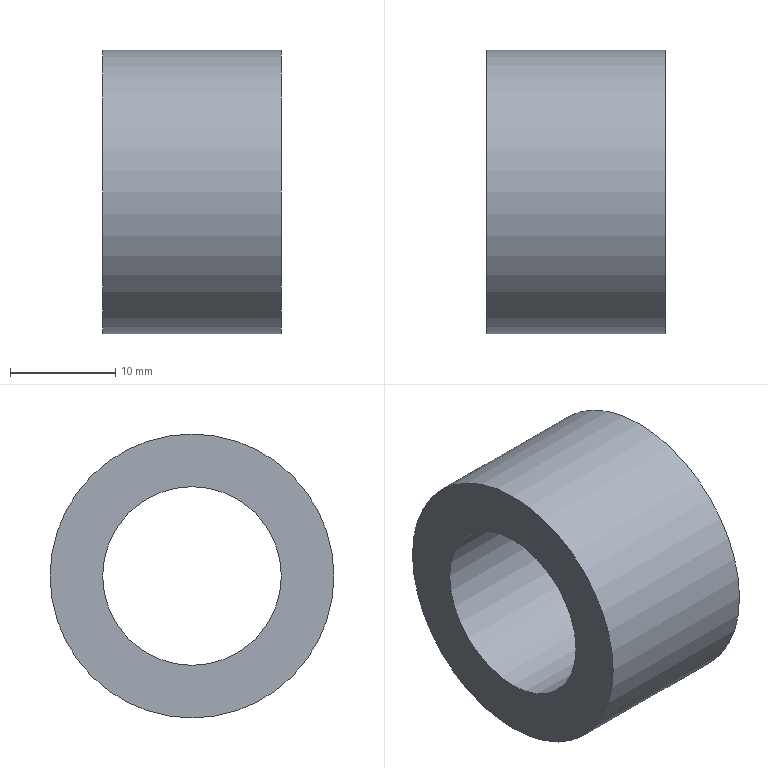Component | NX | SHORT_BUSHING | 1 solid | 4 faces | box 17 x 27 x 27 mm | volume 5875 mm3 | cylinder 2 | plane 2 | commonest cylinder face diameters 27 x1 17 x1
STEP:
#1=CARTESIAN_POINT('',(0.,0.,0.));
#2=DIRECTION('',(0.,0.,1.));
#3=DIRECTION('',(1.,0.,0.));
#4=AXIS2_PLACEMENT_3D('',#1,#2,#3);
#5=CARTESIAN_POINT('',(-2.,0.,109.5));
#6=VERTEX_POINT('',#5);
#7=CARTESIAN_POINT('',(-2.,0.,123.));
#8=DIRECTION('',(-1.,0.,0.));
#9=DIRECTION('',(0.,0.,-1.));
#10=AXIS2_PLACEMENT_3D('',#7,#8,#9);
#11=CIRCLE('',#10,13.5);
#12=CARTESIAN_POINT('',(-2.,0.,123.));
#13=DIRECTION('',(-1.,0.,0.));
#14=DIRECTION('',(0.,0.,1.));
#15=AXIS2_PLACEMENT_3D('',#12,#13,#14);
#16=CYLINDRICAL_SURFACE('',#15,13.5);
#17=CARTESIAN_POINT('',(3.142,0.));
#18=DIRECTION('',(1.,0.));
#19=VECTOR('',#18,1.);
#20=LINE('',#17,#19);
#21=(GEOMETRIC_REPRESENTATION_CONTEXT(2)PARAMETRIC_REPRESENTATION_CONTEXT()REPRESENTATION_CONTEXT('',''));
#22=DEFINITIONAL_REPRESENTATION('',(#20),#21);
#23=PCURVE('',#16,#22);
#24=CARTESIAN_POINT('',(-2.,0.,123.));
#25=DIRECTION('',(-1.,0.,0.));
#26=DIRECTION('',(0.,0.,1.));
#27=AXIS2_PLACEMENT_3D('',#24,#25,#26);
#28=PLANE('',#27);
#29=CARTESIAN_POINT('',(0.,0.));
#30=DIRECTION('',(-1.,0.));
#31=AXIS2_PLACEMENT_2D('',#29,#30);
#32=CIRCLE('',#31,13.5);
#33=(GEOMETRIC_REPRESENTATION_CONTEXT(2)PARAMETRIC_REPRESENTATION_CONTEXT()REPRESENTATION_CONTEXT('',''));
#34=DEFINITIONAL_REPRESENTATION('',(#32),#33);
#35=PCURVE('',#28,#34);
#36=SURFACE_CURVE('',#11,(#23,#35),.PCURVE_S1.);
#37=EDGE_CURVE('',#6,#6,#36,.T.);
#38=ORIENTED_EDGE('',*,*,#37,.T.);
#39=CARTESIAN_POINT('',(-19.,0.,109.5));
#40=VERTEX_POINT('',#39);
#41=CARTESIAN_POINT('',(-2.,0.,109.5));
#42=CARTESIAN_POINT('',(-19.,0.,109.5));
#43=B_SPLINE_CURVE_WITH_KNOTS('',1,(#41,#42),.UNSPECIFIED.,.F.,.F.,(2,2),(0.,17.),.PIECEWISE_BEZIER_KNOTS.);
#44=CARTESIAN_POINT('',(9.425,0.));
#45=DIRECTION('',(0.,1.));
#46=VECTOR('',#45,1.);
#47=LINE('',#44,#46);
#48=(GEOMETRIC_REPRESENTATION_CONTEXT(2)PARAMETRIC_REPRESENTATION_CONTEXT()REPRESENTATION_CONTEXT('',''));
#49=DEFINITIONAL_REPRESENTATION('',(#47),#48);
#50=PCURVE('',#16,#49);
#51=CARTESIAN_POINT('',(3.142,0.));
#52=DIRECTION('',(0.,1.));
#53=VECTOR('',#52,1.);
#54=LINE('',#51,#53);
#55=(GEOMETRIC_REPRESENTATION_CONTEXT(2)PARAMETRIC_REPRESENTATION_CONTEXT()REPRESENTATION_CONTEXT('',''));
#56=DEFINITIONAL_REPRESENTATION('',(#54),#55);
#57=PCURVE('',#16,#56);
#58=SEAM_CURVE('',#43,(#50,#57),.PCURVE_S1.);
#59=EDGE_CURVE('',#6,#40,#58,.T.);
#60=ORIENTED_EDGE('',*,*,#59,.T.);
#61=CARTESIAN_POINT('',(-19.,0.,123.));
#62=DIRECTION('',(-1.,0.,0.));
#63=DIRECTION('',(0.,0.,-1.));
#64=AXIS2_PLACEMENT_3D('',#61,#62,#63);
#65=CIRCLE('',#64,13.5);
#66=CARTESIAN_POINT('',(3.142,17.));
#67=DIRECTION('',(1.,0.));
#68=VECTOR('',#67,1.);
#69=LINE('',#66,#68);
#70=(GEOMETRIC_REPRESENTATION_CONTEXT(2)PARAMETRIC_REPRESENTATION_CONTEXT()REPRESENTATION_CONTEXT('',''));
#71=DEFINITIONAL_REPRESENTATION('',(#69),#70);
#72=PCURVE('',#16,#71);
#73=CARTESIAN_POINT('',(-19.,0.,123.));
#74=DIRECTION('',(-1.,0.,0.));
#75=DIRECTION('',(0.,0.,1.));
#76=AXIS2_PLACEMENT_3D('',#73,#74,#75);
#77=PLANE('',#76);
#78=CARTESIAN_POINT('',(0.,0.));
#79=DIRECTION('',(-1.,0.));
#80=AXIS2_PLACEMENT_2D('',#78,#79);
#81=CIRCLE('',#80,13.5);
#82=(GEOMETRIC_REPRESENTATION_CONTEXT(2)PARAMETRIC_REPRESENTATION_CONTEXT()REPRESENTATION_CONTEXT('',''));
#83=DEFINITIONAL_REPRESENTATION('',(#81),#82);
#84=PCURVE('',#77,#83);
#85=SURFACE_CURVE('',#65,(#72,#84),.PCURVE_S1.);
#86=EDGE_CURVE('',#40,#40,#85,.T.);
#87=ORIENTED_EDGE('',*,*,#86,.F.);
#88=ORIENTED_EDGE('',*,*,#59,.F.);
#89=EDGE_LOOP('',(#38,#60,#87,#88));
#90=FACE_BOUND('',#89,.T.);
#91=ADVANCED_FACE('',(#90),#16,.T.);
#92=CARTESIAN_POINT('',(-2.,0.,114.5));
#93=VERTEX_POINT('',#92);
#94=CARTESIAN_POINT('',(-2.,0.,123.));
#95=DIRECTION('',(-1.,0.,0.));
#96=DIRECTION('',(0.,0.,-1.));
#97=AXIS2_PLACEMENT_3D('',#94,#95,#96);
#98=CIRCLE('',#97,8.5);
#99=CARTESIAN_POINT('',(-2.,0.,123.));
#100=DIRECTION('',(-1.,0.,0.));
#101=DIRECTION('',(0.,0.,1.));
#102=AXIS2_PLACEMENT_3D('',#99,#100,#101);
#103=CYLINDRICAL_SURFACE('',#102,8.5);
#104=CARTESIAN_POINT('',(3.142,0.));
#105=DIRECTION('',(1.,0.));
#106=VECTOR('',#105,1.);
#107=LINE('',#104,#106);
#108=(GEOMETRIC_REPRESENTATION_CONTEXT(2)PARAMETRIC_REPRESENTATION_CONTEXT()REPRESENTATION_CONTEXT('',''));
#109=DEFINITIONAL_REPRESENTATION('',(#107),#108);
#110=PCURVE('',#103,#109);
#111=CARTESIAN_POINT('',(0.,0.));
#112=DIRECTION('',(-1.,0.));
#113=AXIS2_PLACEMENT_2D('',#111,#112);
#114=CIRCLE('',#113,8.5);
#115=(GEOMETRIC_REPRESENTATION_CONTEXT(2)PARAMETRIC_REPRESENTATION_CONTEXT()REPRESENTATION_CONTEXT('',''));
#116=DEFINITIONAL_REPRESENTATION('',(#114),#115);
#117=PCURVE('',#28,#116);
#118=SURFACE_CURVE('',#98,(#110,#117),.PCURVE_S1.);
#119=EDGE_CURVE('',#93,#93,#118,.T.);
#120=ORIENTED_EDGE('',*,*,#119,.T.);
#121=CARTESIAN_POINT('',(-19.,0.,114.5));
#122=VERTEX_POINT('',#121);
#123=CARTESIAN_POINT('',(-2.,0.,114.5));
#124=CARTESIAN_POINT('',(-19.,0.,114.5));
#125=B_SPLINE_CURVE_WITH_KNOTS('',1,(#123,#124),.UNSPECIFIED.,.F.,.F.,(2,2),(0.,17.),.PIECEWISE_BEZIER_KNOTS.);
#126=CARTESIAN_POINT('',(9.425,0.));
#127=DIRECTION('',(0.,1.));
#128=VECTOR('',#127,1.);
#129=LINE('',#126,#128);
#130=(GEOMETRIC_REPRESENTATION_CONTEXT(2)PARAMETRIC_REPRESENTATION_CONTEXT()REPRESENTATION_CONTEXT('',''));
#131=DEFINITIONAL_REPRESENTATION('',(#129),#130);
#132=PCURVE('',#103,#131);
#133=CARTESIAN_POINT('',(3.142,0.));
#134=DIRECTION('',(0.,1.));
#135=VECTOR('',#134,1.);
#136=LINE('',#133,#135);
#137=(GEOMETRIC_REPRESENTATION_CONTEXT(2)PARAMETRIC_REPRESENTATION_CONTEXT()REPRESENTATION_CONTEXT('',''));
#138=DEFINITIONAL_REPRESENTATION('',(#136),#137);
#139=PCURVE('',#103,#138);
#140=SEAM_CURVE('',#125,(#132,#139),.PCURVE_S1.);
#141=EDGE_CURVE('',#93,#122,#140,.T.);
#142=ORIENTED_EDGE('',*,*,#141,.T.);
#143=CARTESIAN_POINT('',(-19.,0.,123.));
#144=DIRECTION('',(-1.,0.,0.));
#145=DIRECTION('',(0.,0.,-1.));
#146=AXIS2_PLACEMENT_3D('',#143,#144,#145);
#147=CIRCLE('',#146,8.5);
#148=CARTESIAN_POINT('',(3.142,17.));
#149=DIRECTION('',(1.,0.));
#150=VECTOR('',#149,1.);
#151=LINE('',#148,#150);
#152=(GEOMETRIC_REPRESENTATION_CONTEXT(2)PARAMETRIC_REPRESENTATION_CONTEXT()REPRESENTATION_CONTEXT('',''));
#153=DEFINITIONAL_REPRESENTATION('',(#151),#152);
#154=PCURVE('',#103,#153);
#155=CARTESIAN_POINT('',(0.,0.));
#156=DIRECTION('',(-1.,0.));
#157=AXIS2_PLACEMENT_2D('',#155,#156);
#158=CIRCLE('',#157,8.5);
#159=(GEOMETRIC_REPRESENTATION_CONTEXT(2)PARAMETRIC_REPRESENTATION_CONTEXT()REPRESENTATION_CONTEXT('',''));
#160=DEFINITIONAL_REPRESENTATION('',(#158),#159);
#161=PCURVE('',#77,#160);
#162=SURFACE_CURVE('',#147,(#154,#161),.PCURVE_S1.);
#163=EDGE_CURVE('',#122,#122,#162,.T.);
#164=ORIENTED_EDGE('',*,*,#163,.F.);
#165=ORIENTED_EDGE('',*,*,#141,.F.);
#166=EDGE_LOOP('',(#120,#142,#164,#165));
#167=FACE_BOUND('',#166,.F.);
#168=ADVANCED_FACE('',(#167),#103,.F.);
#169=ORIENTED_EDGE('',*,*,#37,.F.);
#170=EDGE_LOOP('',(#169));
#171=FACE_BOUND('',#170,.T.);
#172=ORIENTED_EDGE('',*,*,#119,.T.);
#173=EDGE_LOOP('',(#172));
#174=FACE_BOUND('',#173,.T.);
#175=ADVANCED_FACE('',(#171,#174),#28,.F.);
#176=ORIENTED_EDGE('',*,*,#86,.T.);
#177=EDGE_LOOP('',(#176));
#178=FACE_BOUND('',#177,.T.);
#179=ORIENTED_EDGE('',*,*,#163,.F.);
#180=EDGE_LOOP('',(#179));
#181=FACE_BOUND('',#180,.T.);
#182=ADVANCED_FACE('',(#178,#181),#77,.T.);
#183=CLOSED_SHELL('',(#91,#168,#175,#182));
#184=MANIFOLD_SOLID_BREP('',#183);
#185=(LENGTH_UNIT()NAMED_UNIT(*)SI_UNIT(.MILLI.,.METRE.));
#186=UNCERTAINTY_MEASURE_WITH_UNIT(LENGTH_MEASURE(0.00001),#185,'','');
#187=(NAMED_UNIT(*)PLANE_ANGLE_UNIT()SI_UNIT($,.RADIAN.));
#188=(NAMED_UNIT(*)SI_UNIT($,.STERADIAN.)SOLID_ANGLE_UNIT());
#189=(GEOMETRIC_REPRESENTATION_CONTEXT(3)GLOBAL_UNCERTAINTY_ASSIGNED_CONTEXT((#186))GLOBAL_UNIT_ASSIGNED_CONTEXT((#185,#187,#188))REPRESENTATION_CONTEXT('',''));
#190=ADVANCED_BREP_SHAPE_REPRESENTATION('',(#4,#184),#189);